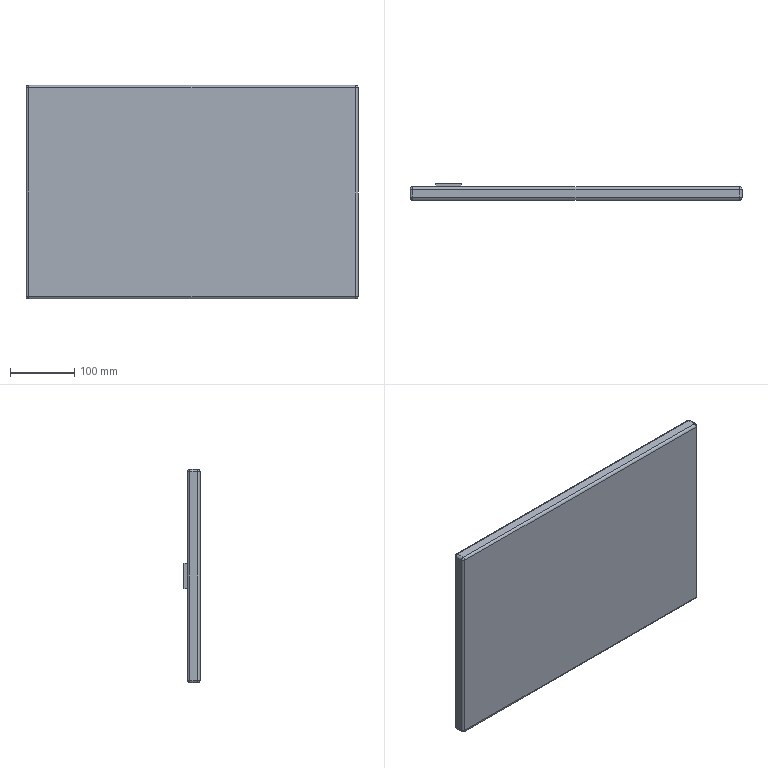Component | SolidWorks | AX00-100.1.1-1_21.1.1-1 | 1 solid | 36 faces | box 518 x 25 x 333 mm | volume 3440223 mm3 | plane 16 | cylinder 12 | sphere 8 | commonest cylinder face diameters 8 x12
build123d program:
from build123d import *

# Parameters (mm, degrees)
SKETCH1_W           = 518
SKETCH1_H           = 333
BOSS_EXTRUDE1_DEPTH = 10
FILLET1_R           = 4
FILLET2_R           = 4
SKETCH2_W           = 40
SKETCH2_H           = 40
SKETCH2_W_2         = 34
SKETCH2_H_2         = 34
BOSS_EXTRUDE2_DEPTH = 5


with BuildPart() as part:
    # Sketch1 → Boss-Extrude1 (new, symmetric)
    with BuildSketch(Plane.XY):
        Rectangle(SKETCH1_W, SKETCH1_H)
    extrude(amount=BOSS_EXTRUDE1_DEPTH, both=True)

    # Fillet1
    fillet1_edges = [part.edges().sort_by_distance(p)[0] for p in [
        (259, -166.5, 0),
        (-259, -166.5, 0),
        (-259, 166.5, 0),
        (259, 166.5, 0),
    ]]
    fillet(fillet1_edges, radius=FILLET1_R)

    # Fillet2
    fillet2_edges = [part.edges().sort_by_distance(p)[0] for p in [
        (0, -166.5, -10),
        (0, -166.5, 10),
        (259, 0, -10),
        (-259, 0, -10),
        (0, 166.5, -10),
        (257.828, 165.328, -10),
        (257.828, -165.328, -10),
        (-257.828, 165.328, -10),
        (-257.828, -165.328, -10),
        (-259, 0, 10),
        (259, 0, 10),
        (0, 166.5, 10),
        (257.828, 165.328, 10),
        (257.828, -165.328, 10),
        (-257.828, 165.328, 10),
        (-257.828, -165.328, 10),
    ]]
    fillet(fillet2_edges, radius=FILLET2_R)

    # Sketch2 → Boss-Extrude2 (add)
    with BuildSketch(Plane.XY.offset(10)):
        with Locations((199, 0)):
            Rectangle(SKETCH2_W, SKETCH2_H)
        with Locations((199, 0)):
            Rectangle(SKETCH2_W_2, SKETCH2_H_2, mode=Mode.SUBTRACT)
    extrude(amount=BOSS_EXTRUDE2_DEPTH)


solid = part.part

# Placed as in the assembly
solid = solid.moved(Location((858.631, 1503.364, -5), (-90, 0, 180)))